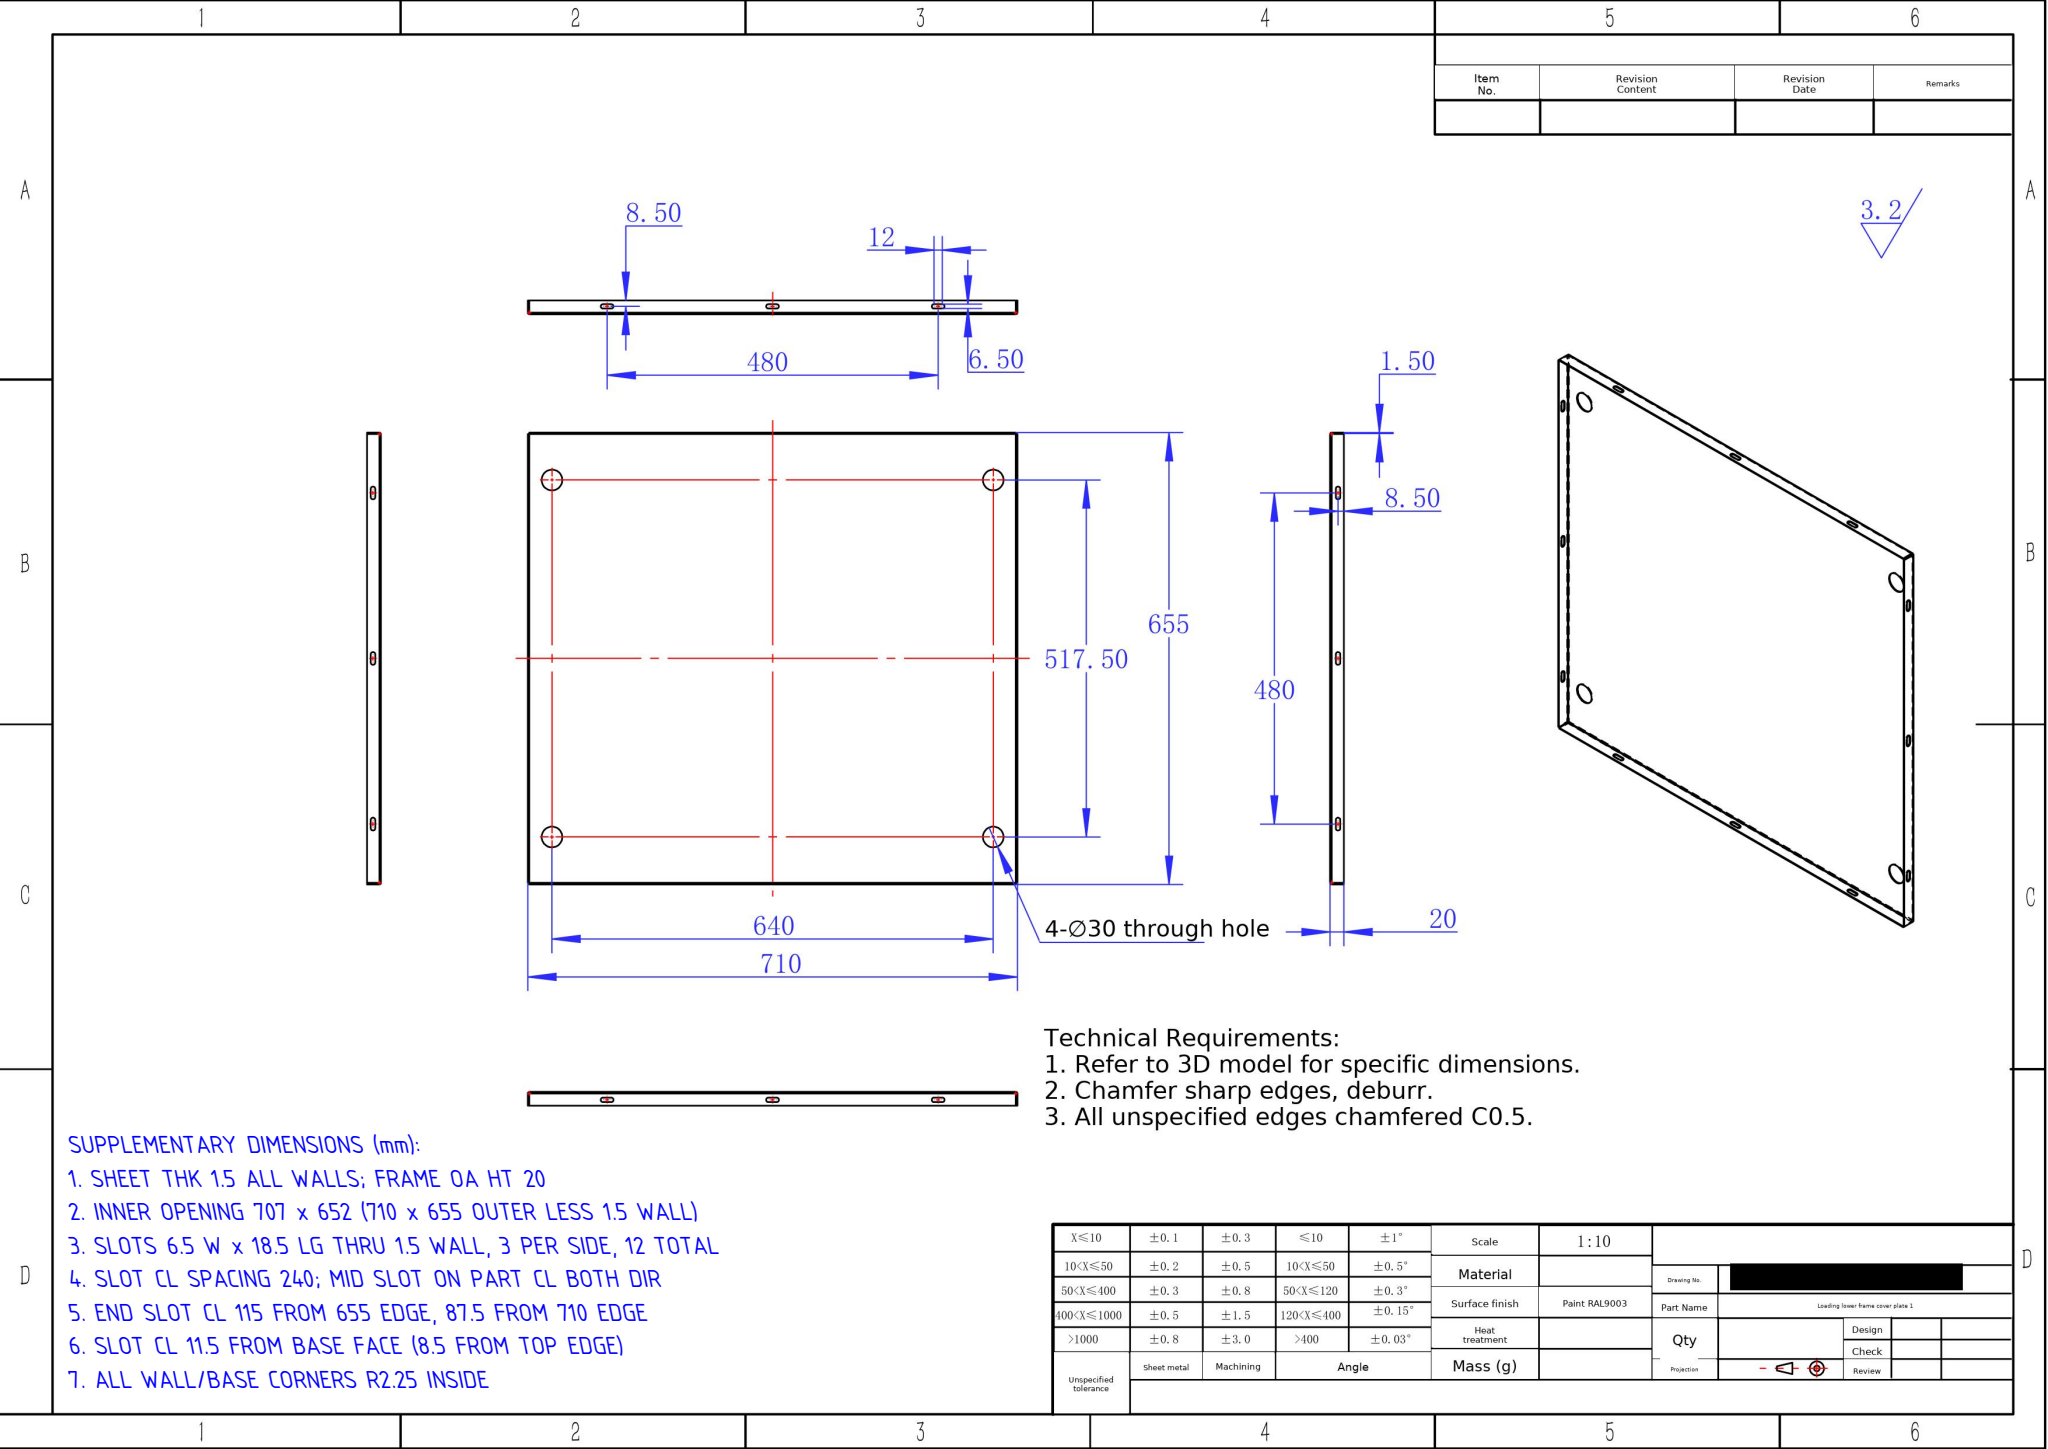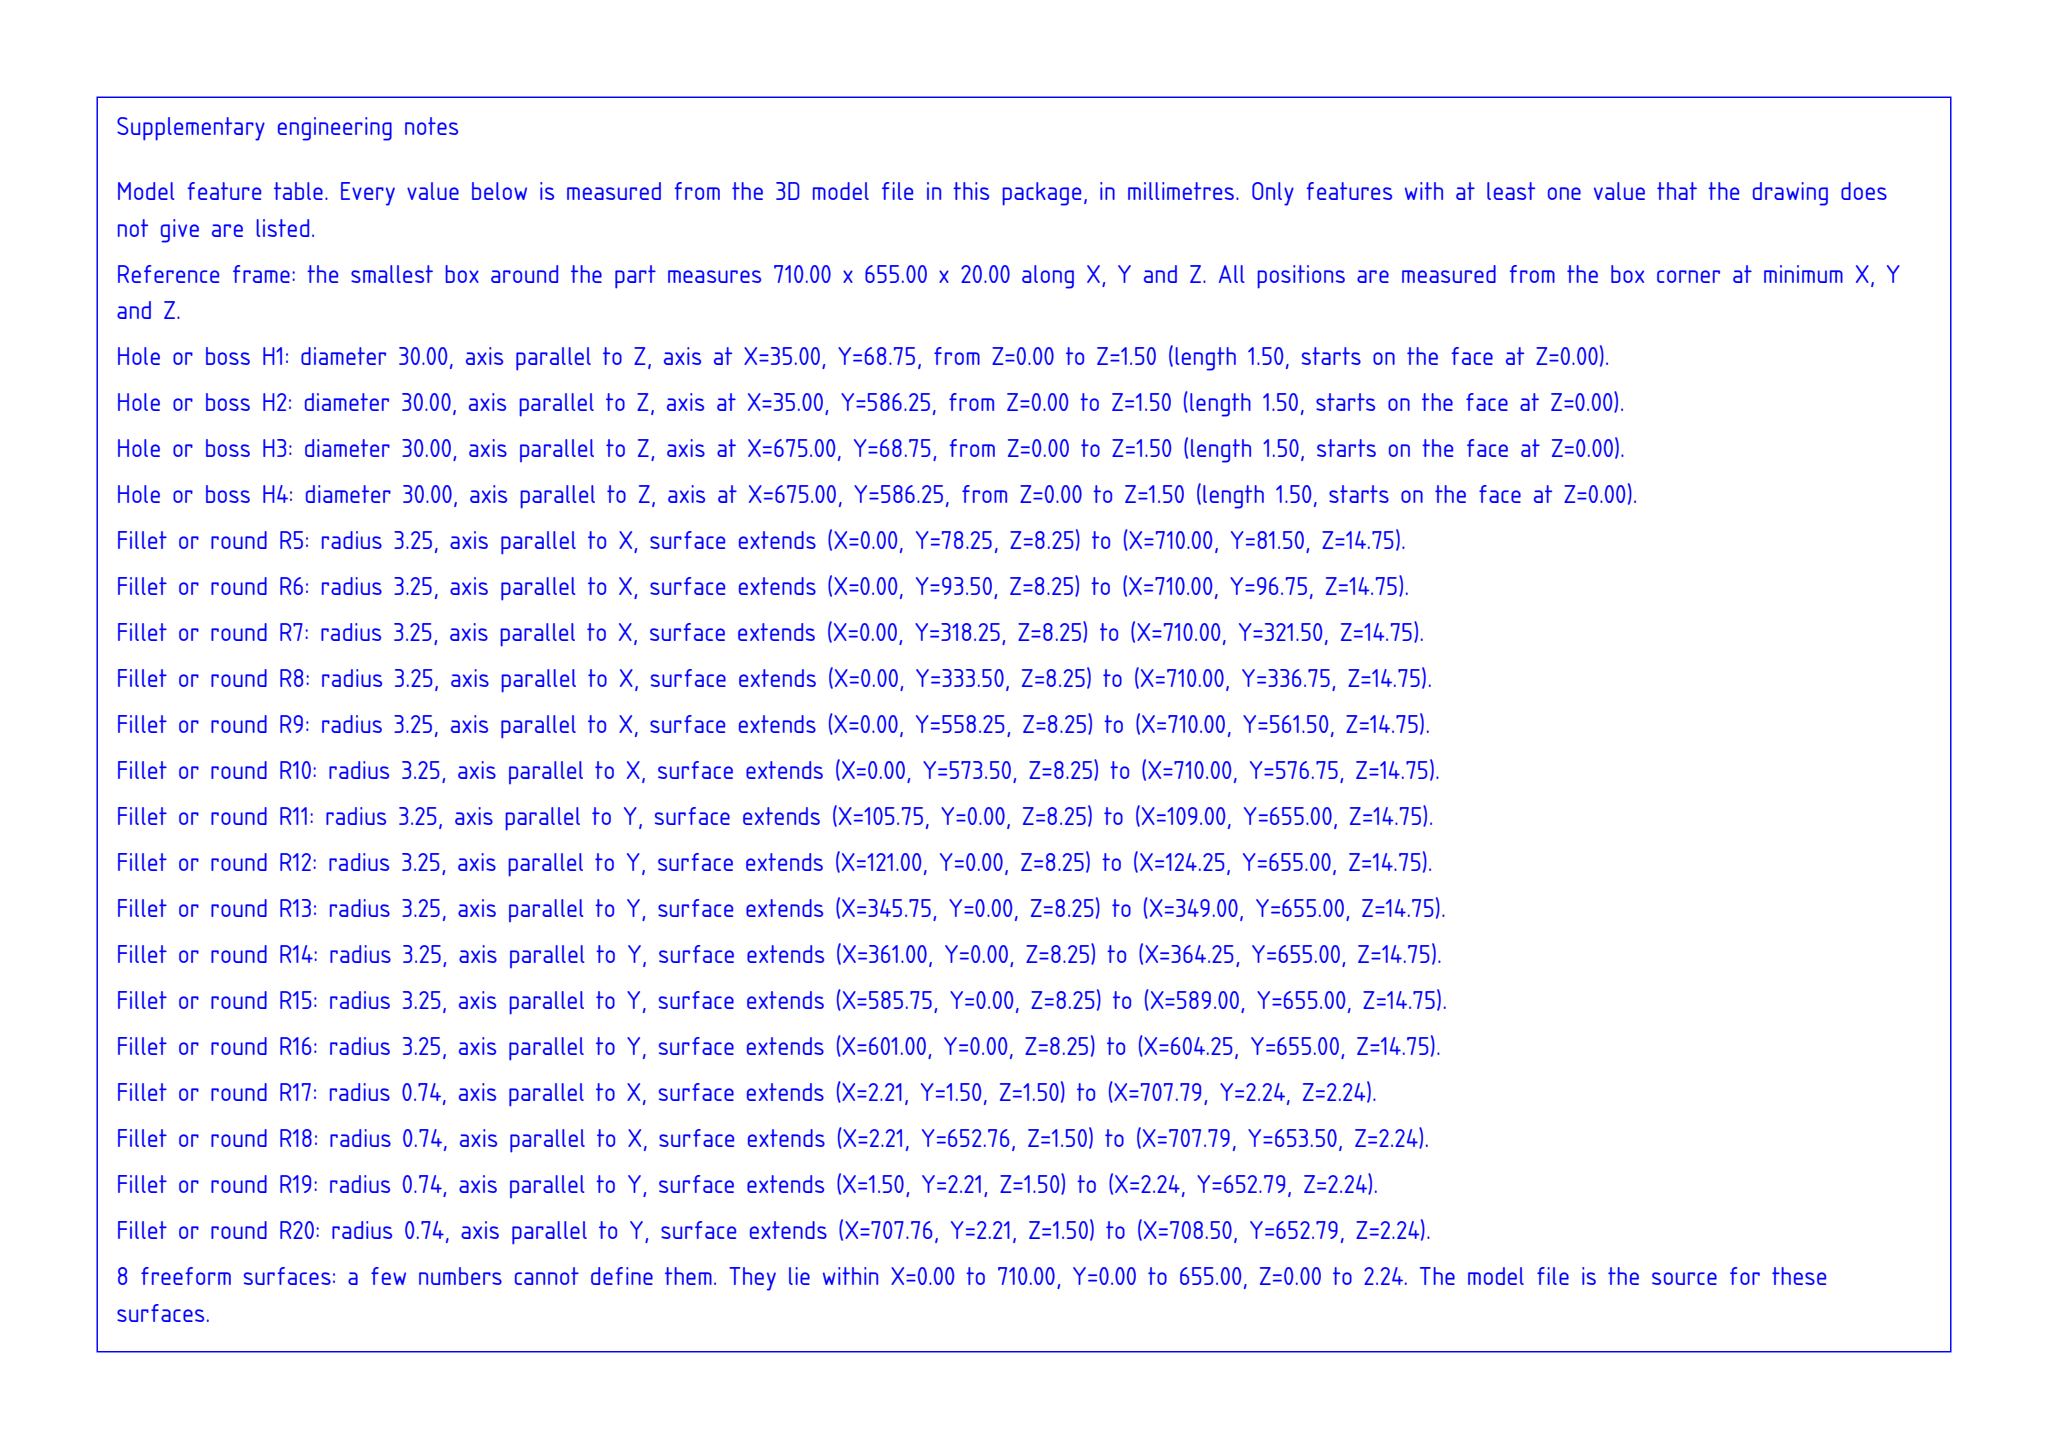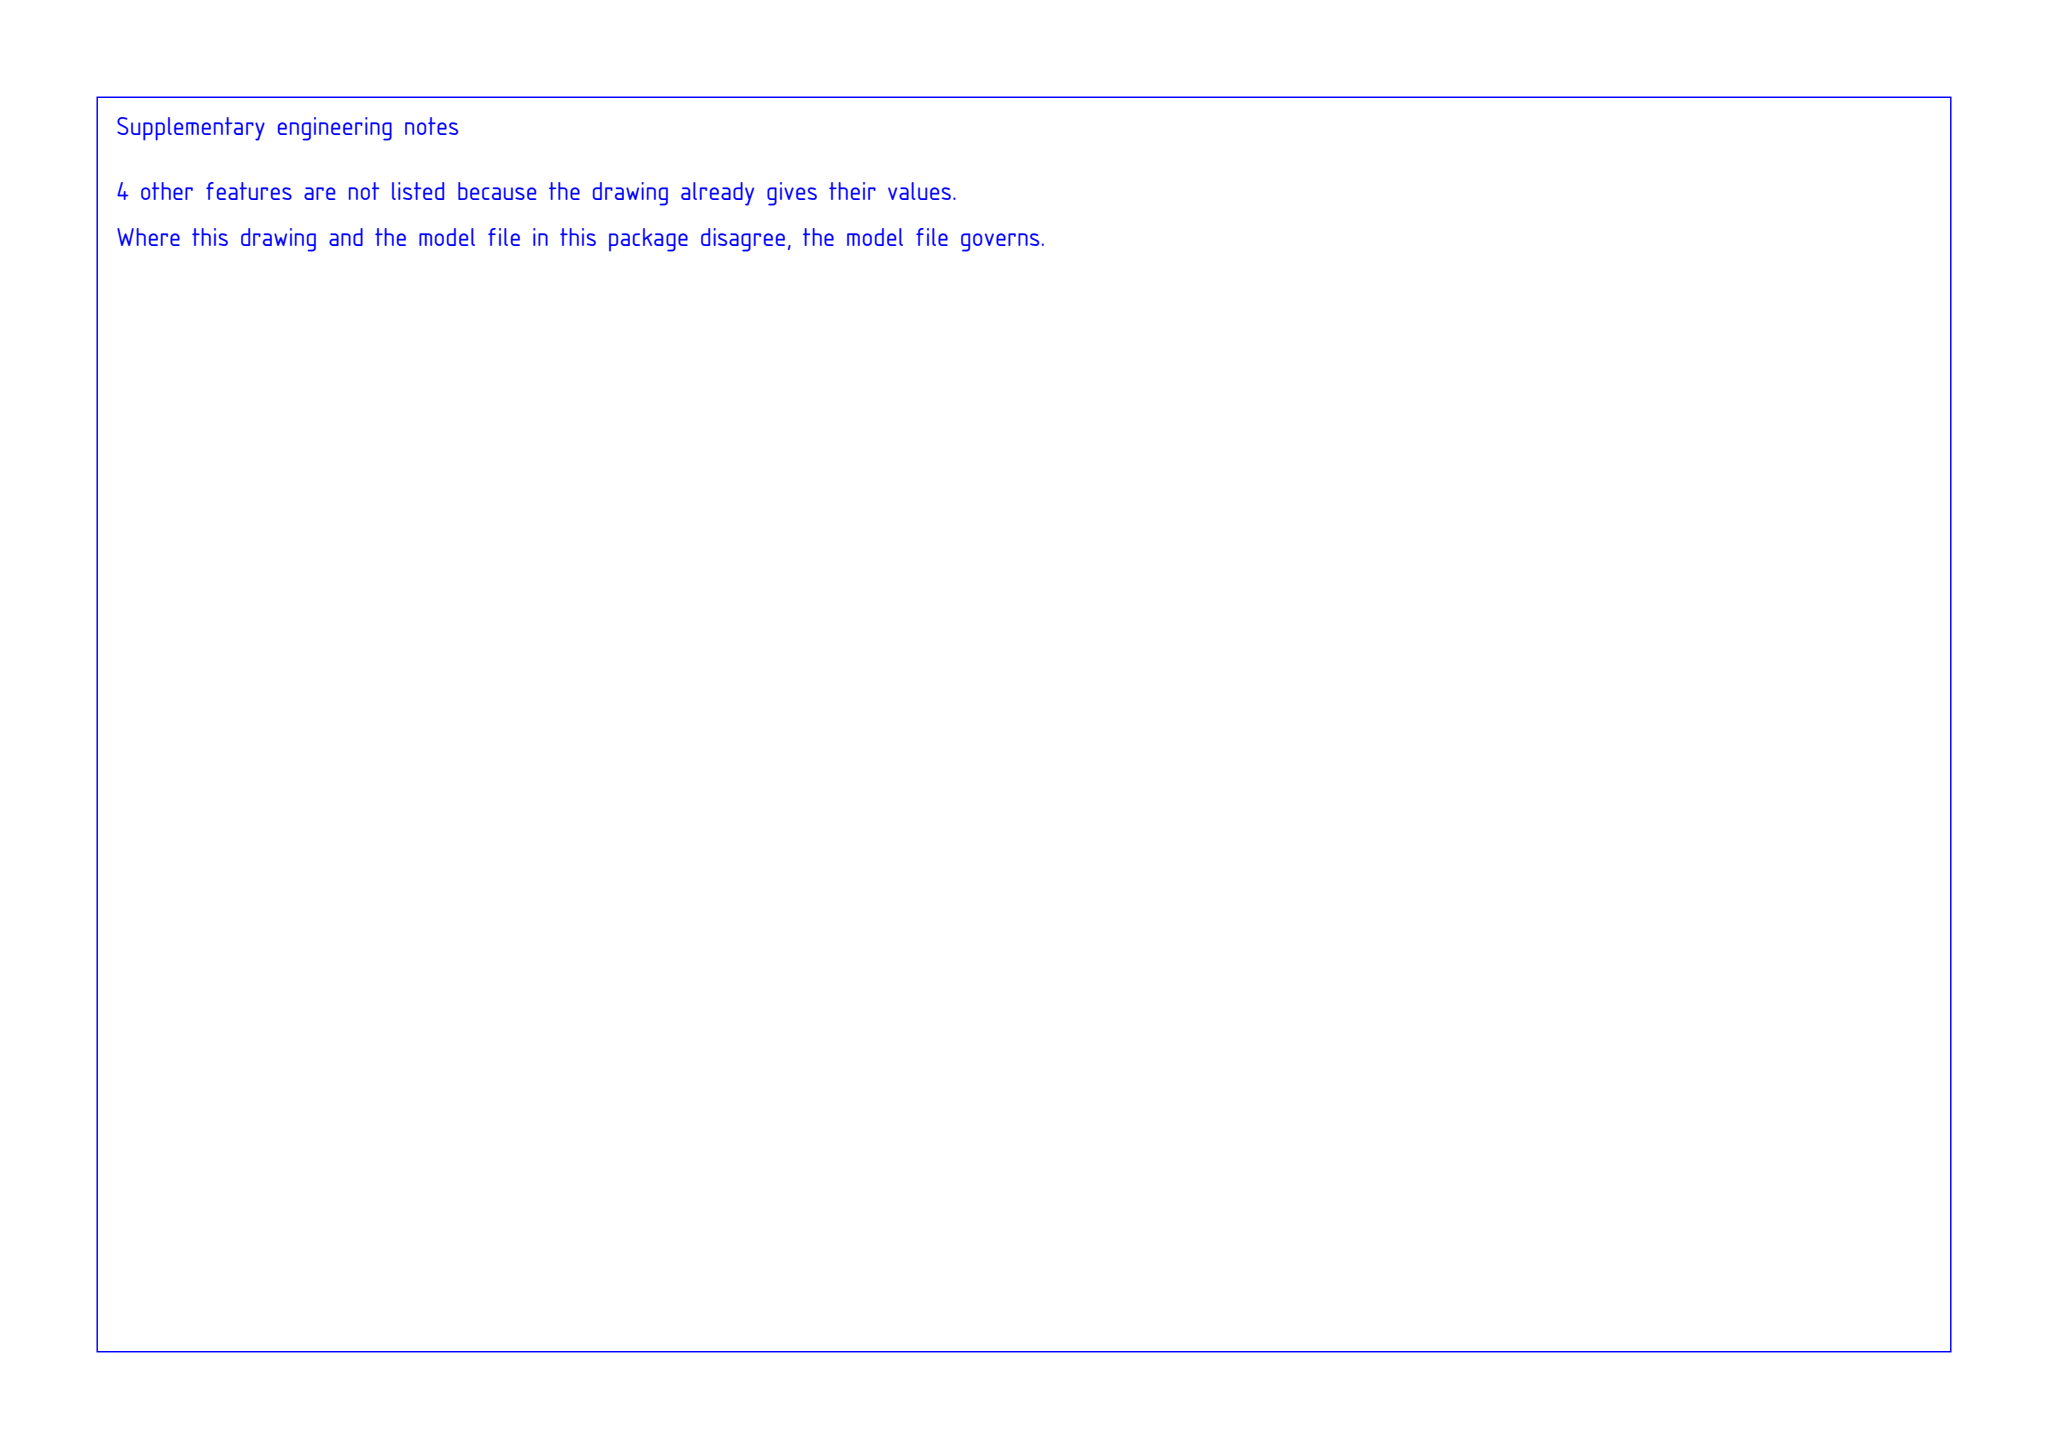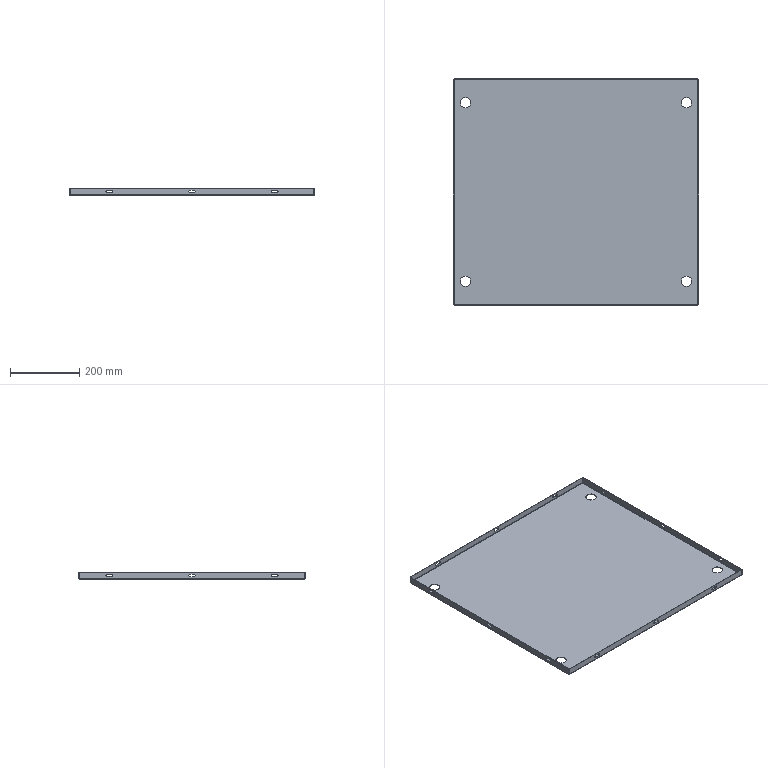Part | SolidWorks | mm | 1 solid | 94 faces | box 710 x 655 x 20 mm | volume 763975 mm3 | plane 46 | cylinder 40 | spline 8 | commonest cylinder face diameters 6.5 x24 30 x8 4.473 x4 1.473 x4